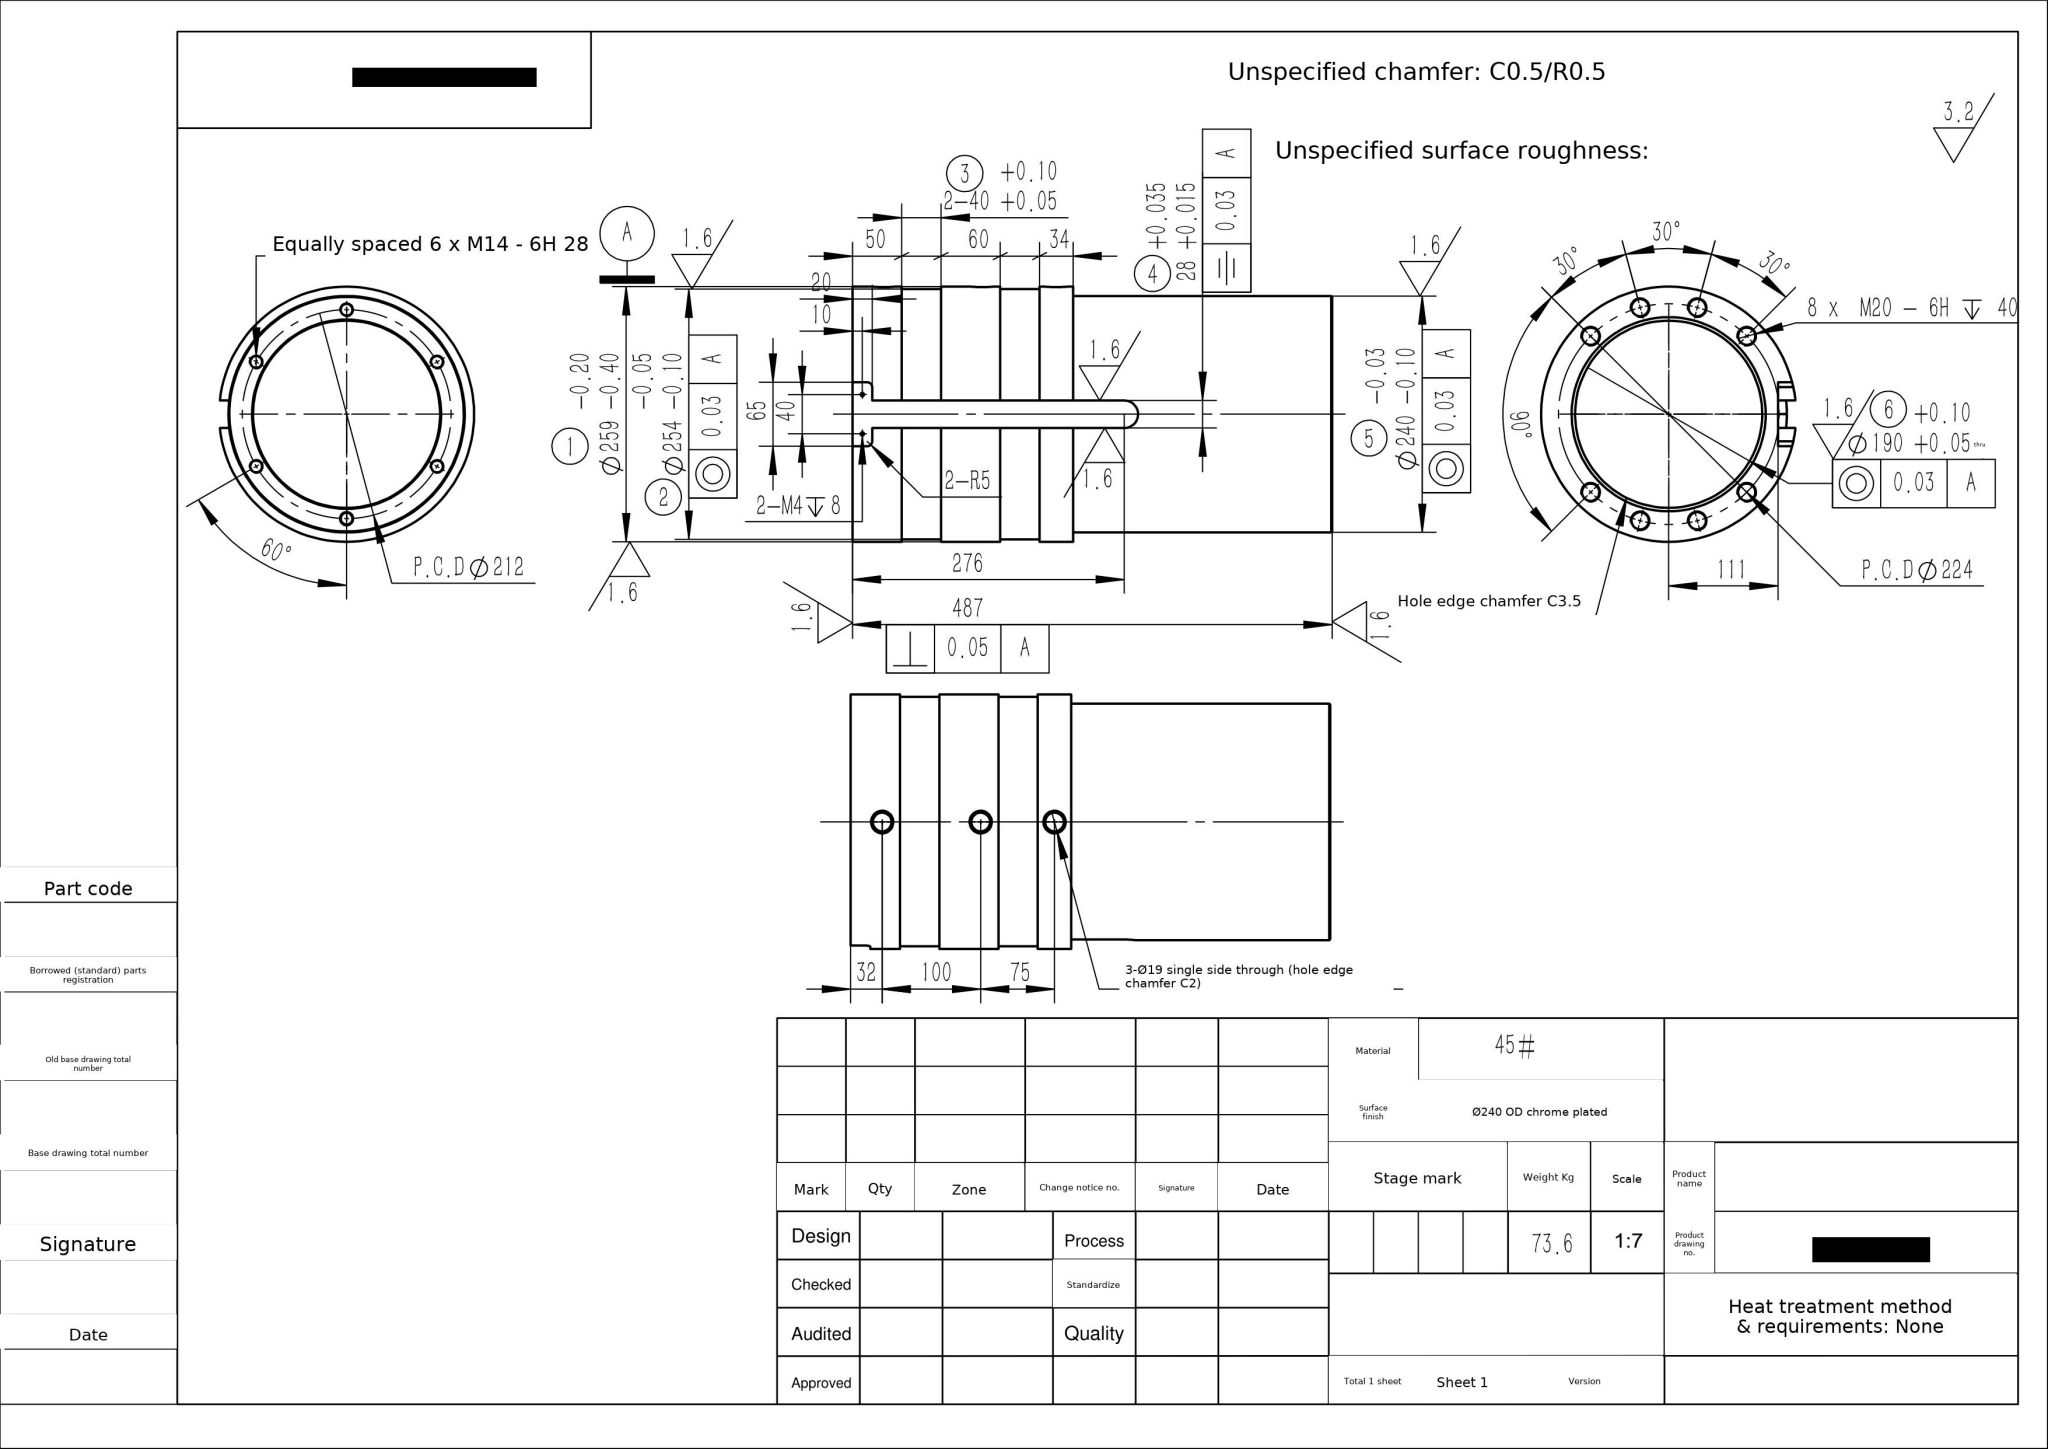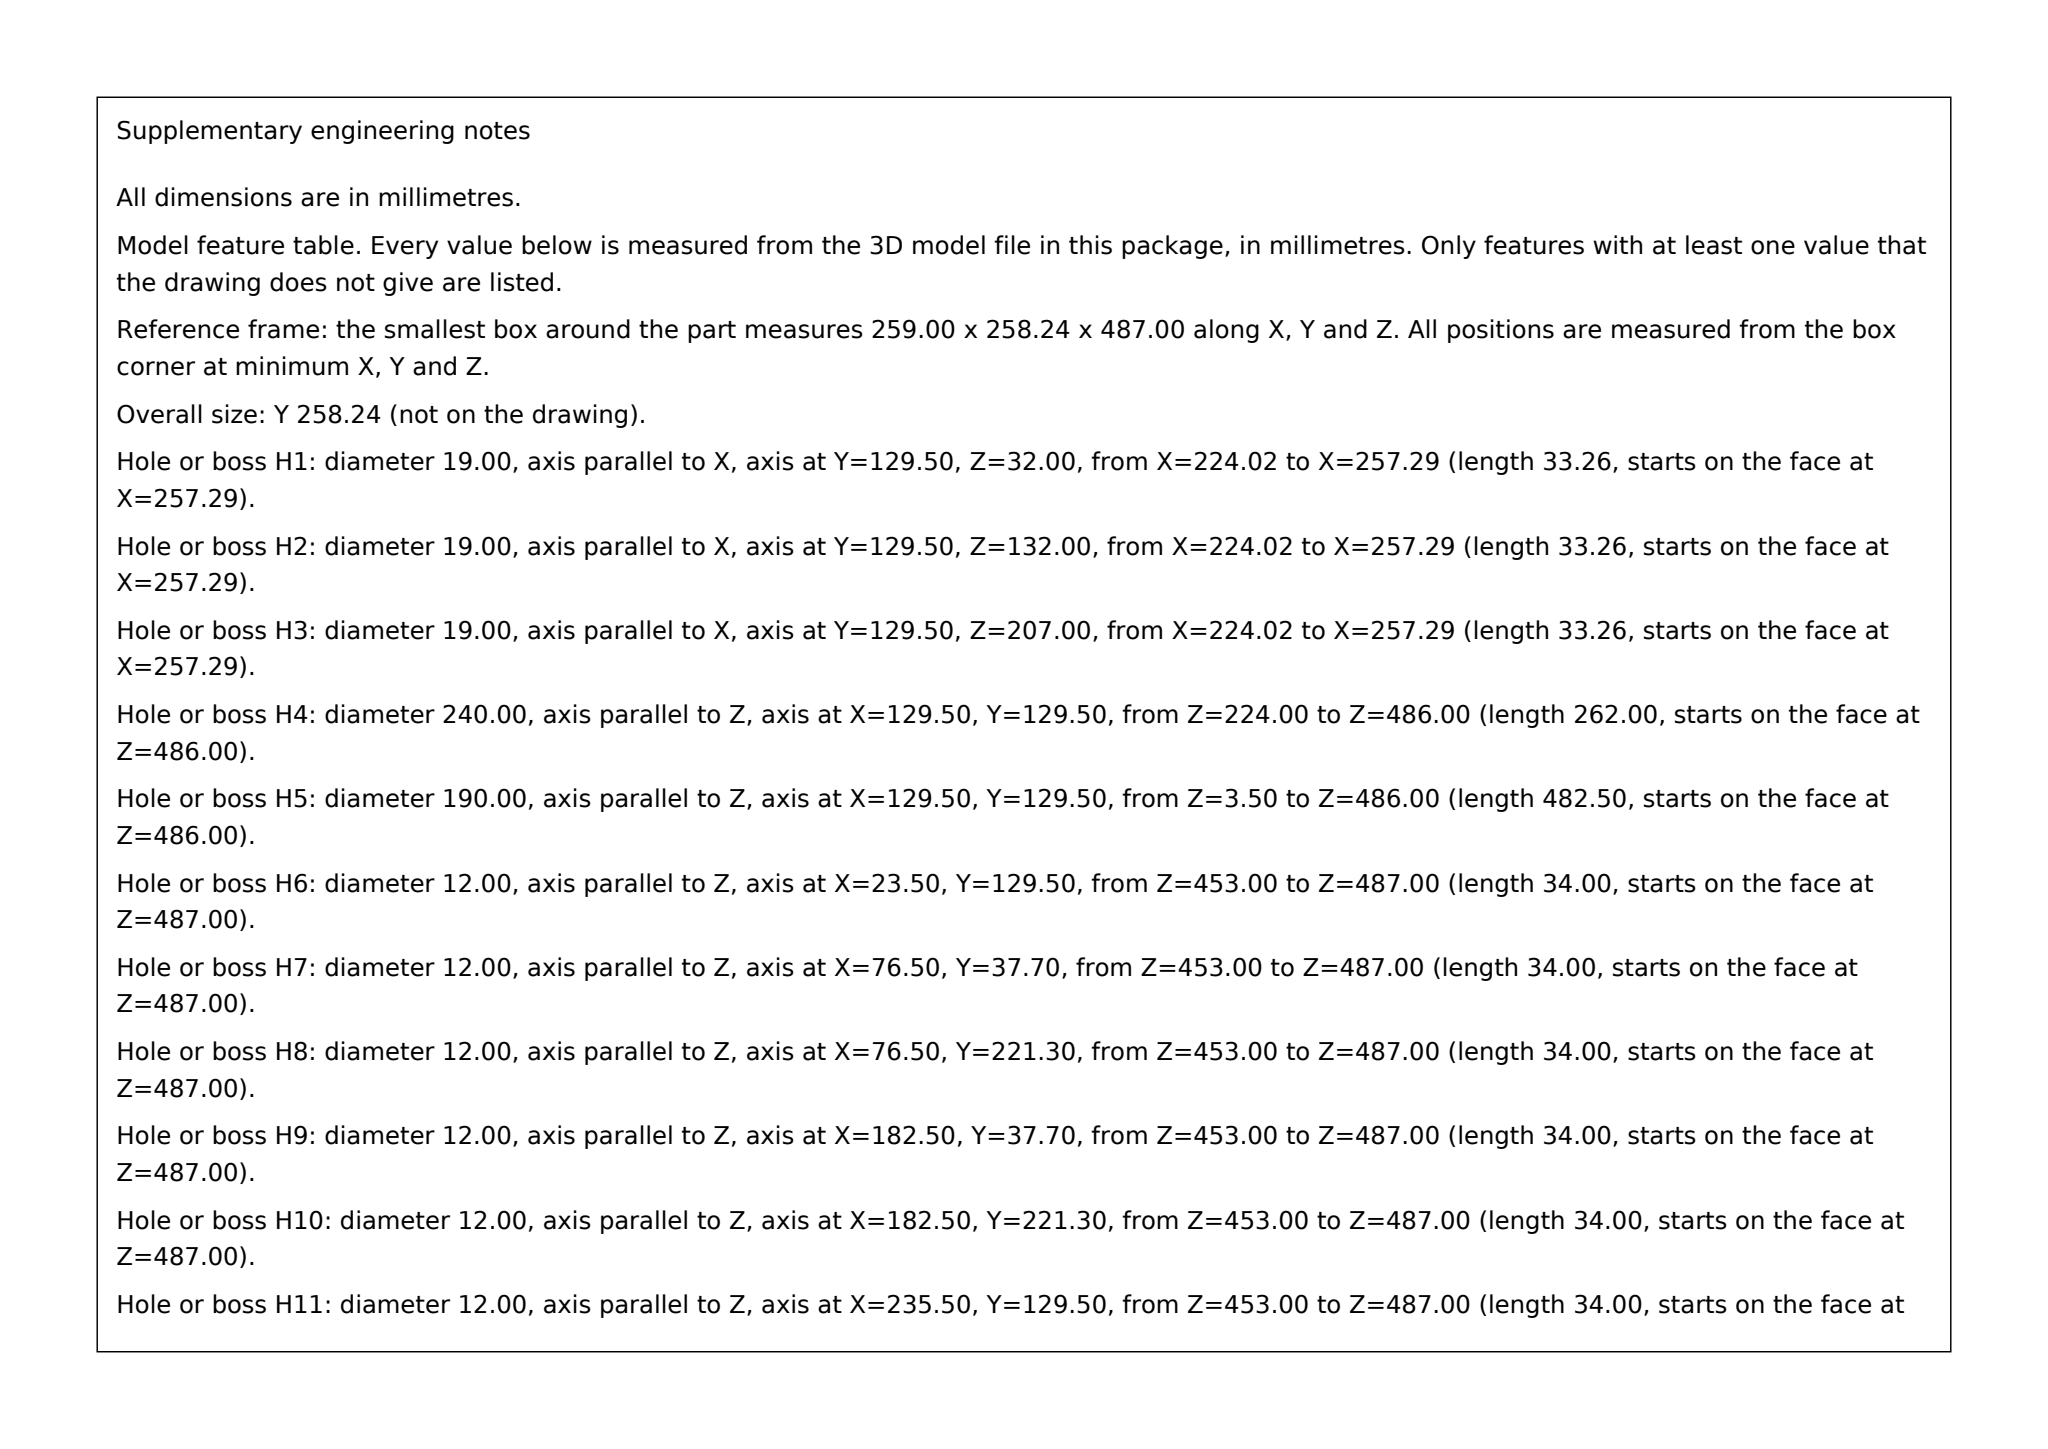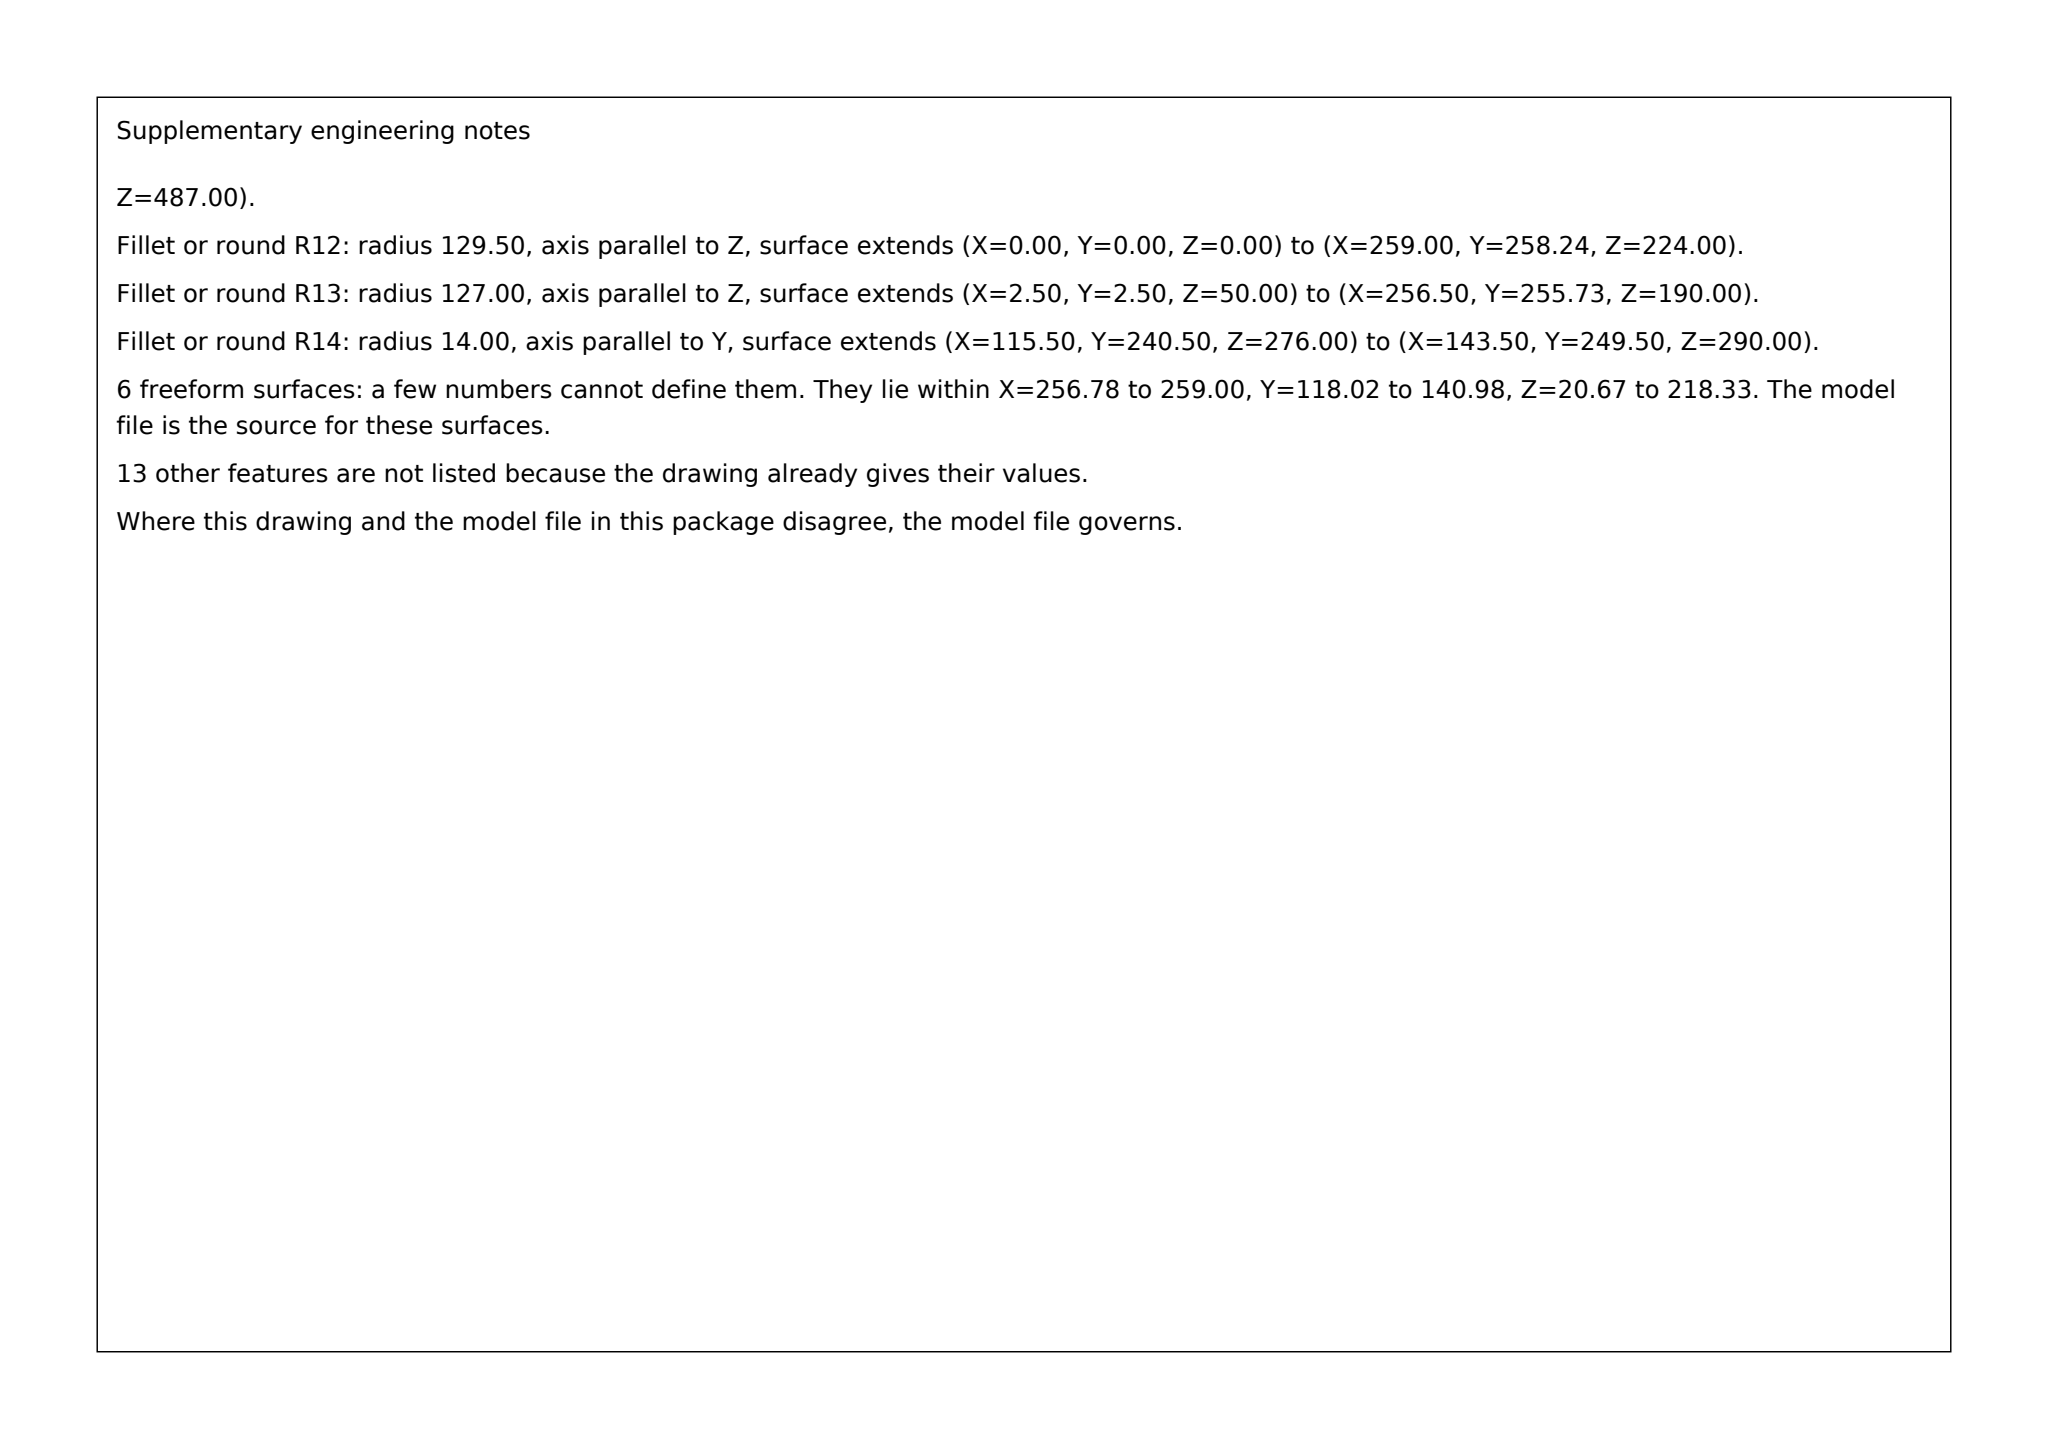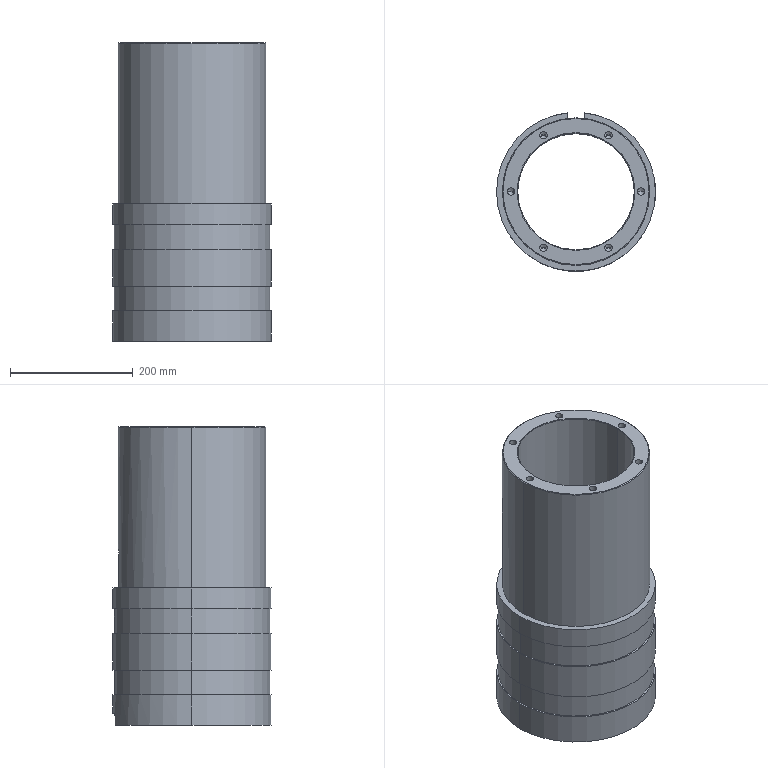Part | SolidWorks | mm | material 45# | 1 solid | 119 faces | box 259 x 258.24 x 487 mm | volume 9441276 mm3 | cylinder 61 | cone 38 | plane 14 | spline 6 | commonest cylinder face diameters 17.5 x16 12 x12 259 x9 19 x6 254 x6 3.3 x4 240 x2 190 x2